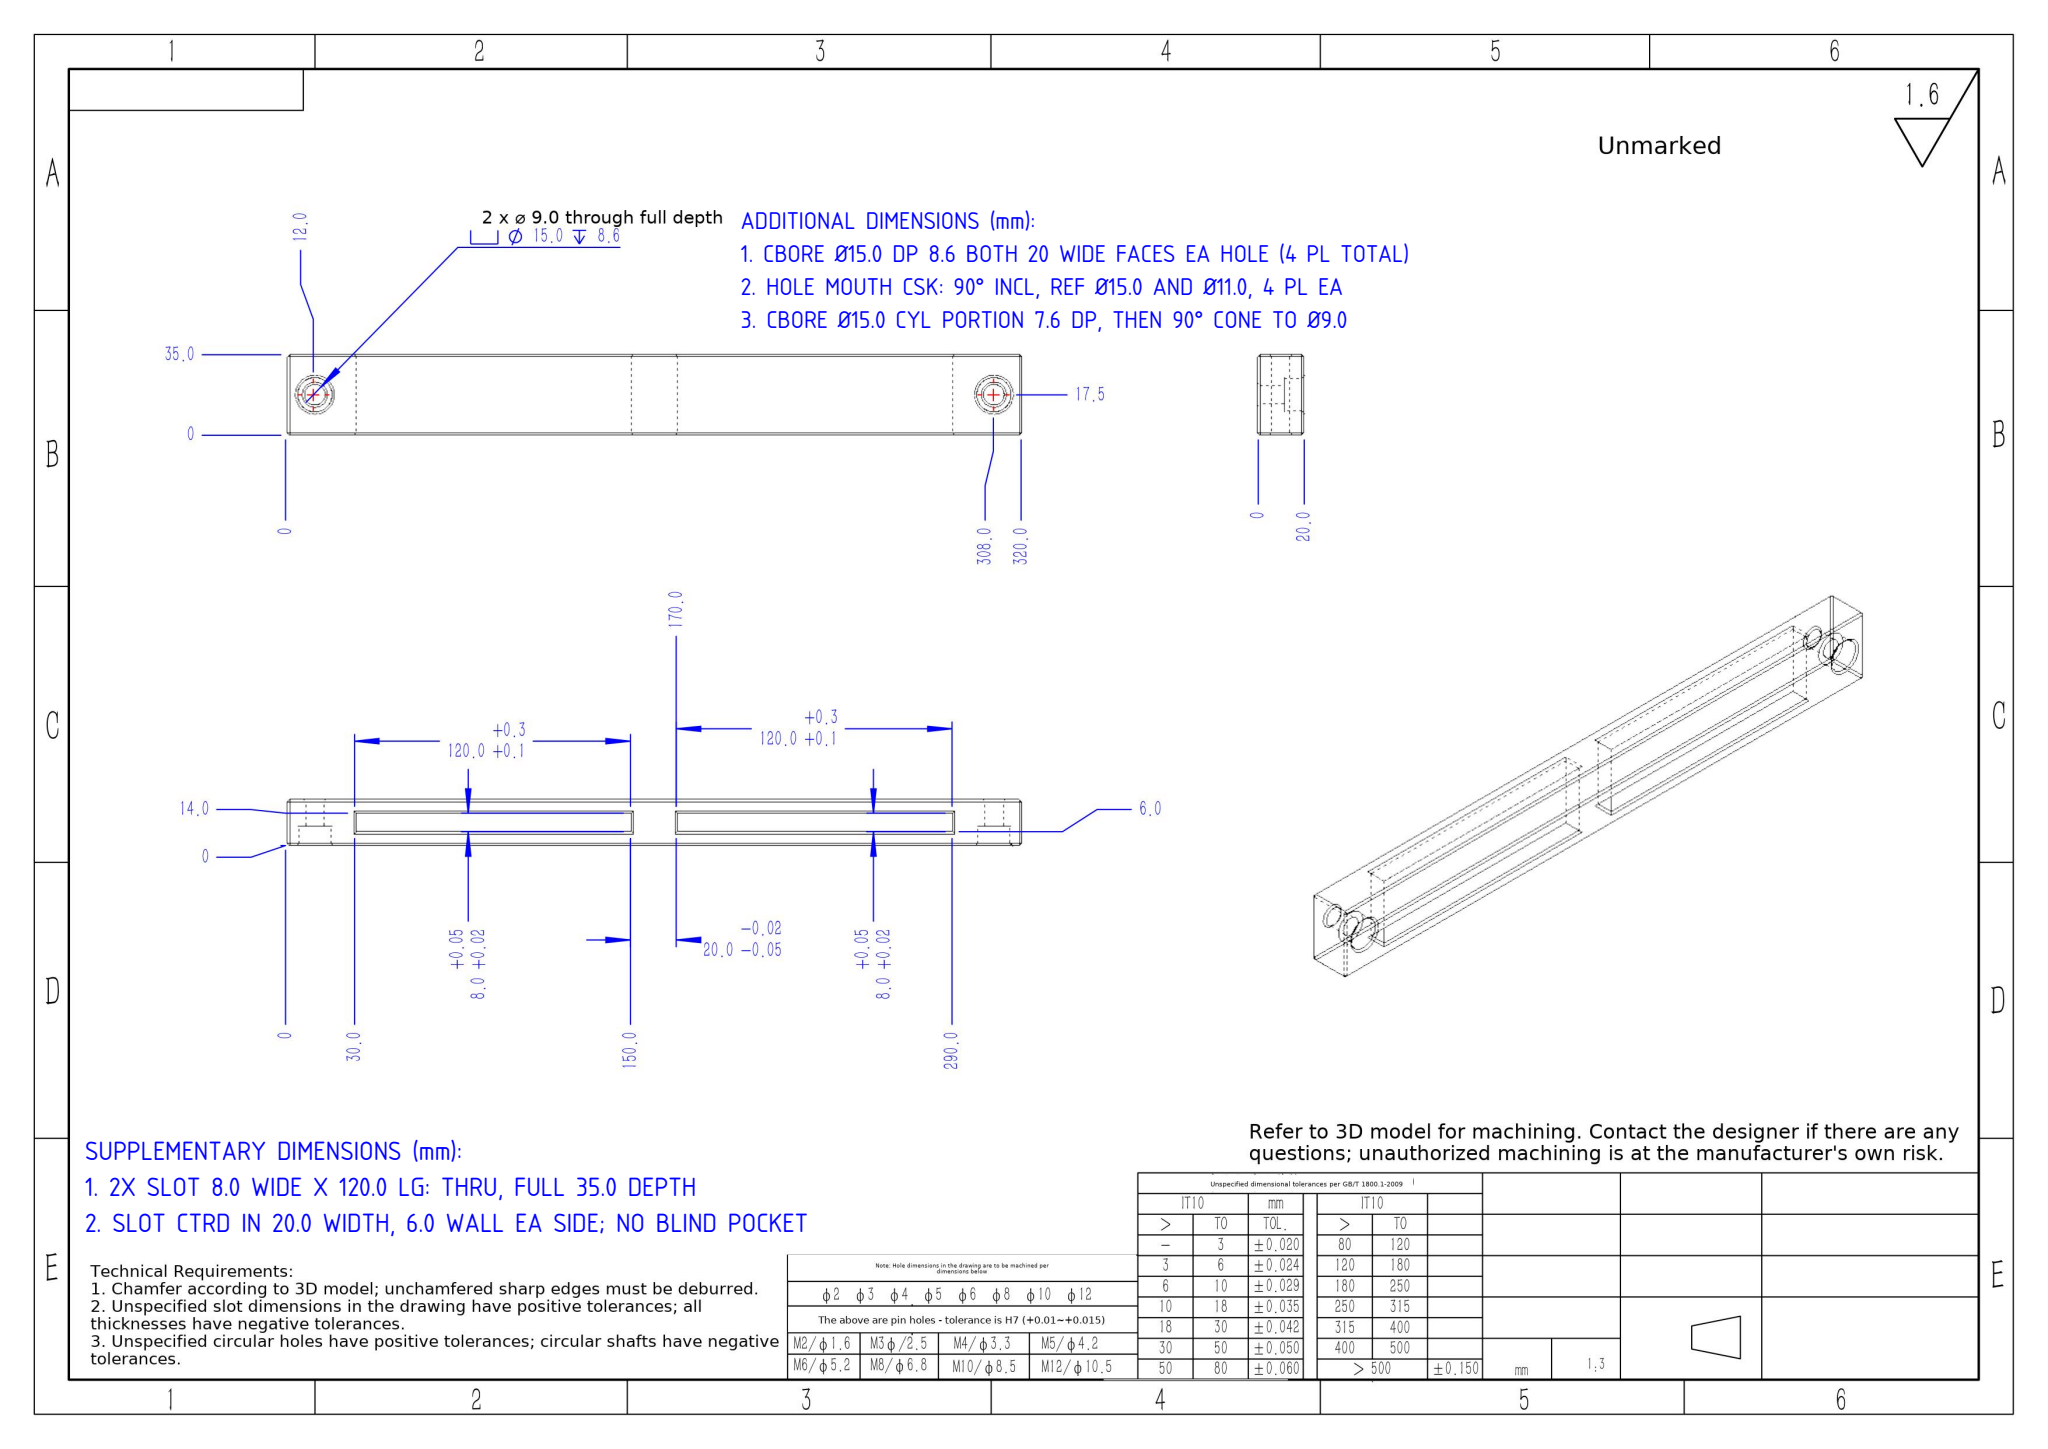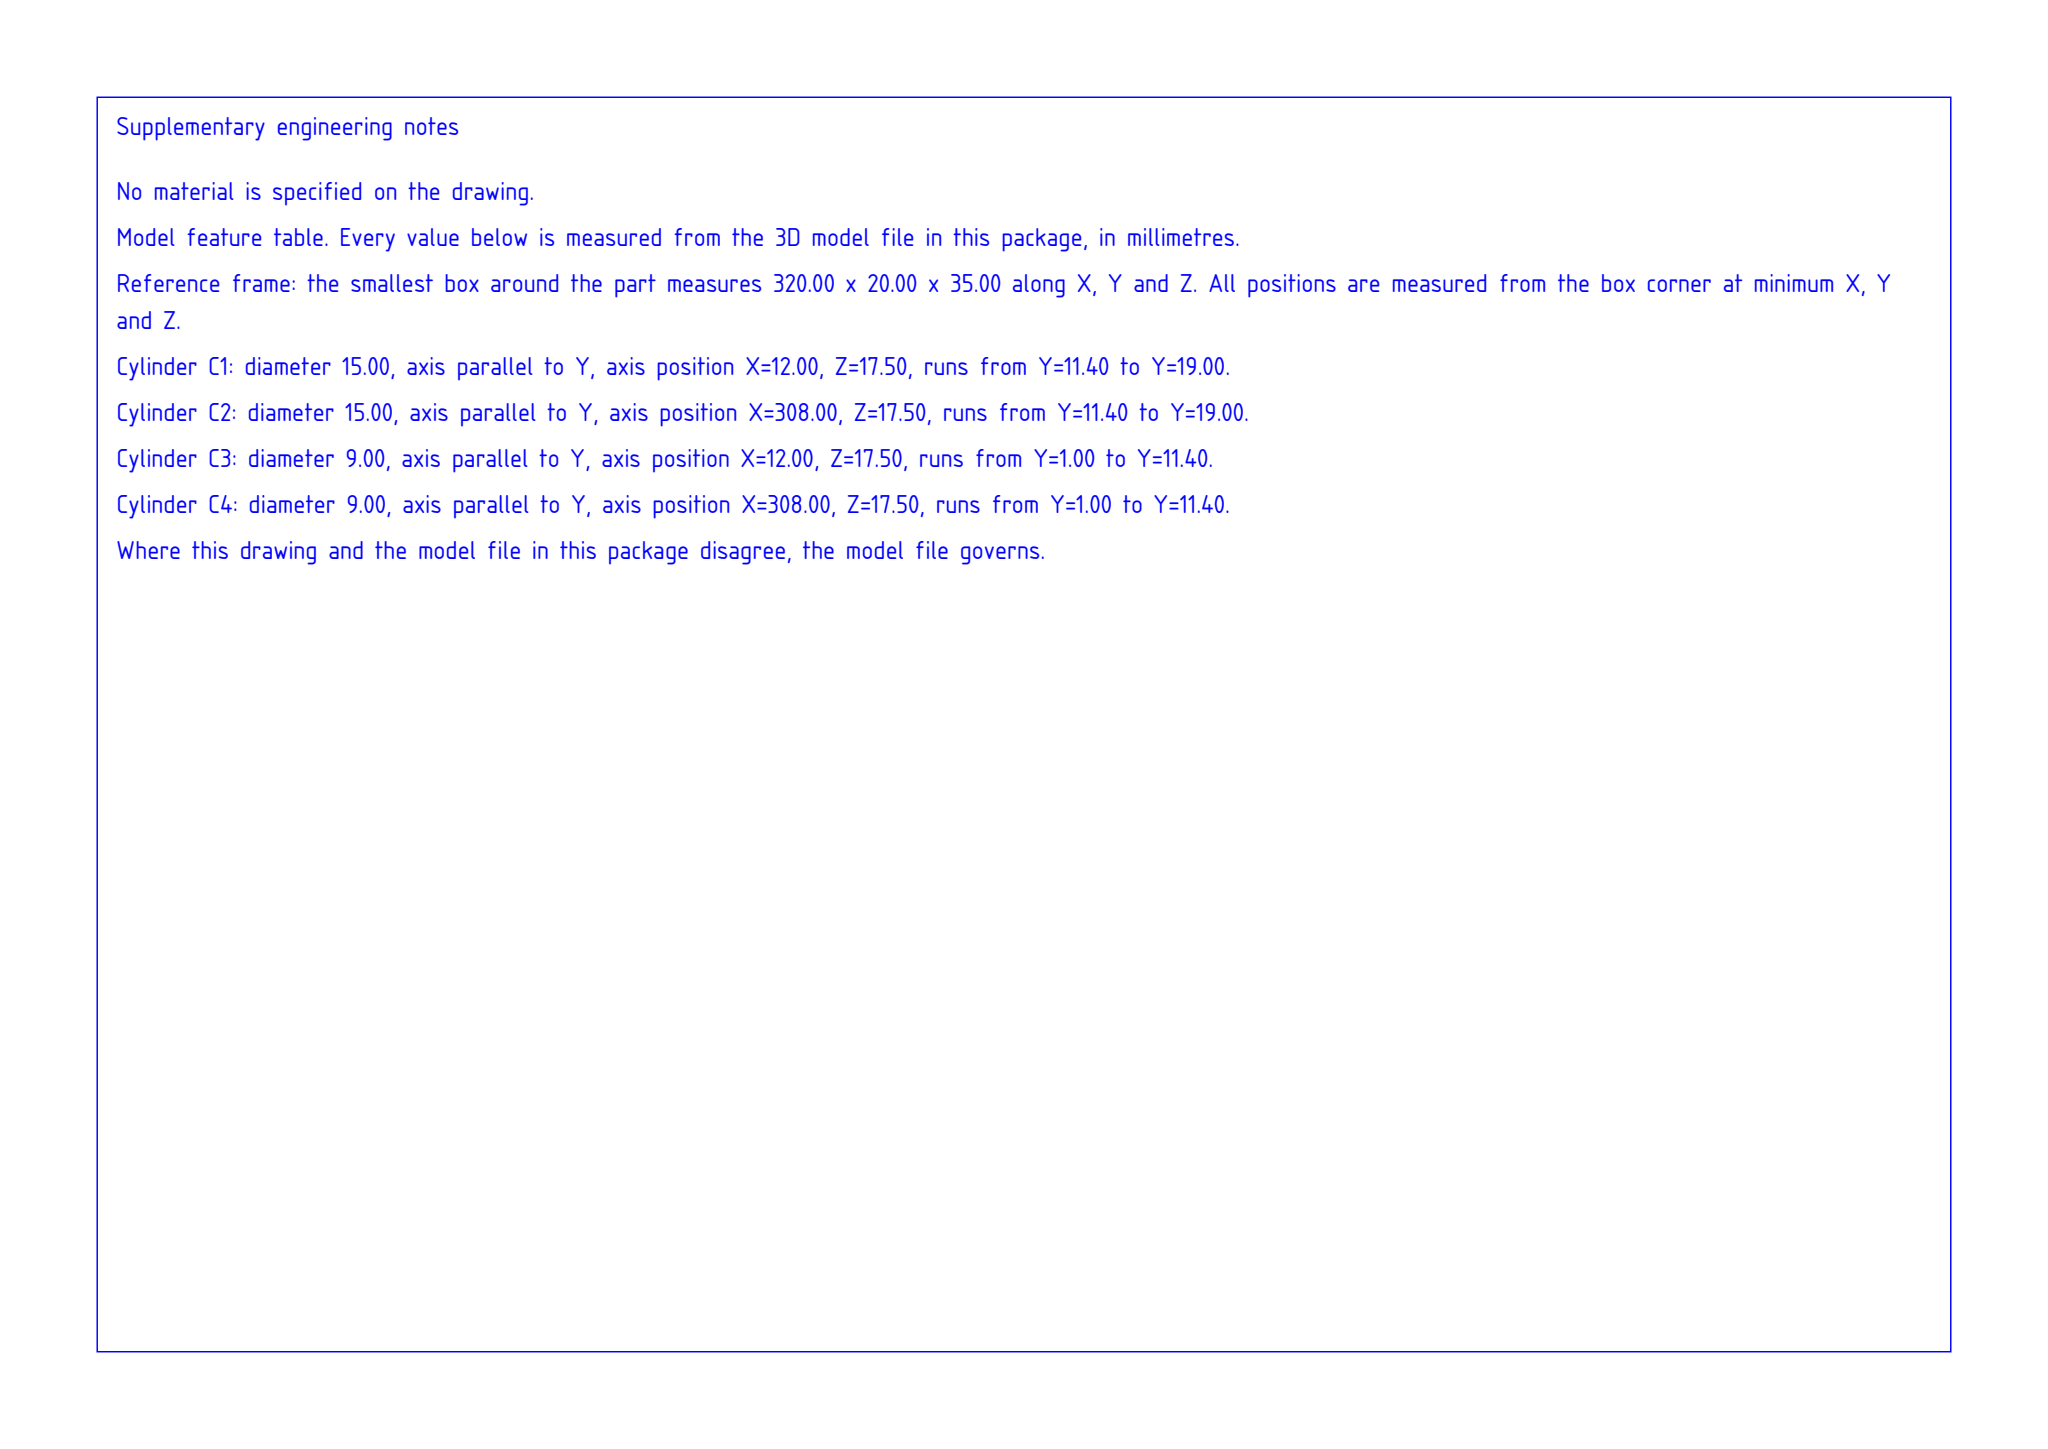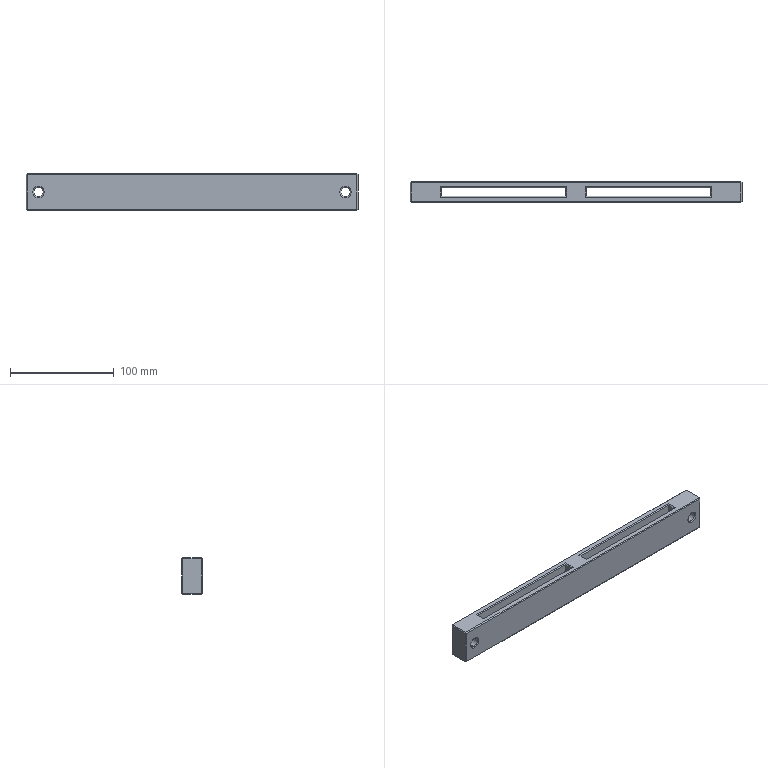Part | SolidWorks | mm | 1 solid | 68 faces | box 320 x 20 x 35 mm | volume 150968 mm3 | plane 52 | cone 8 | cylinder 8 | commonest cylinder face diameters 15 x4 9 x4
build123d program:
from build123d import *

# Parameters (mm, degrees)
SKETCH1_W                                       = 320
SKETCH1_H                                       = 20
BOSS_EXTRUDE1_DEPTH                             = 17.5
M8_HEX_SOCKET_HEAD_CAP_SCREW_CBORE1_D           = 9
M8_HEX_SOCKET_HEAD_CAP_SCREW_CBORE1_CBORE_D     = 15
M8_HEX_SOCKET_HEAD_CAP_SCREW_CBORE1_CBORE_DEPTH = 8.6
SKETCH4_W                                       = 120
SKETCH4_H                                       = 8
CUT_EXTRUDE1_DEPTH                              = 53
CHAMFER2_SIZE                                   = 1


with BuildPart() as part:
    # Sketch1 → Boss-Extrude1 (new, symmetric)
    with BuildSketch(Plane.XY):
        Rectangle(SKETCH1_W, SKETCH1_H)
    extrude(amount=BOSS_EXTRUDE1_DEPTH, both=True)

    # M8 Hex Socket Head Cap Screw CBORE1 (through all)
    with Locations(Plane(origin=(0, 10, 0), x_dir=(1, 0, 0), z_dir=(0, 1, 0))):
        with Locations((148, 0)):
            m8_hex_socket_head_cap_screw_cbore1 = CounterBoreHole(M8_HEX_SOCKET_HEAD_CAP_SCREW_CBORE1_D / 2, M8_HEX_SOCKET_HEAD_CAP_SCREW_CBORE1_CBORE_D / 2, M8_HEX_SOCKET_HEAD_CAP_SCREW_CBORE1_CBORE_DEPTH)

    # Mirror1: M8 Hex Socket Head Cap Screw CBORE1 across plane
    add(m8_hex_socket_head_cap_screw_cbore1.mirror(Plane(origin=(0, 0, 0), x_dir=(0, 0, 1), z_dir=(1, 0, 0))), mode=Mode.SUBTRACT)

    # Sketch4 → Cut-Extrude1 (cut)
    with BuildSketch(Plane(origin=(0, 0, -17.5), x_dir=(-1, 0, 0), z_dir=(0, 0, -1))):
        with Locations((-70, 0)):
            Rectangle(SKETCH4_W, SKETCH4_H)
    cut_extrude1 = extrude(amount=-CUT_EXTRUDE1_DEPTH, mode=Mode.SUBTRACT)

    # Mirror2: Cut-Extrude1 across plane
    add(cut_extrude1.mirror(Plane(origin=(0, 0, 0), x_dir=(0, 0, 1), z_dir=(1, 0, 0))), mode=Mode.SUBTRACT)

    # Chamfer2
    chamfer2_edges = [part.edges().sort_by_distance(p)[0] for p in [
        (-160, 0, 17.5),
        (0, -10, 17.5),
        (140.5, 10, 0),
        (152.5, -10, 0),
        (-140.5, 10, 0),
        (-152.5, -10, 0),
        (10, 0, 17.5),
        (70, -4, 17.5),
        (130, 0, 17.5),
        (70, 4, 17.5),
        (10, 0, -17.5),
        (70, 4, -17.5),
        (130, 0, -17.5),
        (70, -4, -17.5),
        (160, 0, 17.5),
        (0, -10, -17.5),
        (-160, 0, -17.5),
        (-10, 0, -17.5),
        (-70, 4, -17.5),
        (0, 10, -17.5),
        (-130, 0, -17.5),
        (-70, -4, -17.5),
        (-10, 0, 17.5),
        (-70, 4, 17.5),
        (-130, 0, 17.5),
        (-70, -4, 17.5),
        (160, 0, -17.5),
        (0, 10, 17.5),
        (160, -10, 0),
        (-160, -10, 0),
        (-160, 10, 0),
        (160, 10, 0),
    ]]
    chamfer(chamfer2_edges, length=CHAMFER2_SIZE)


solid = part.part